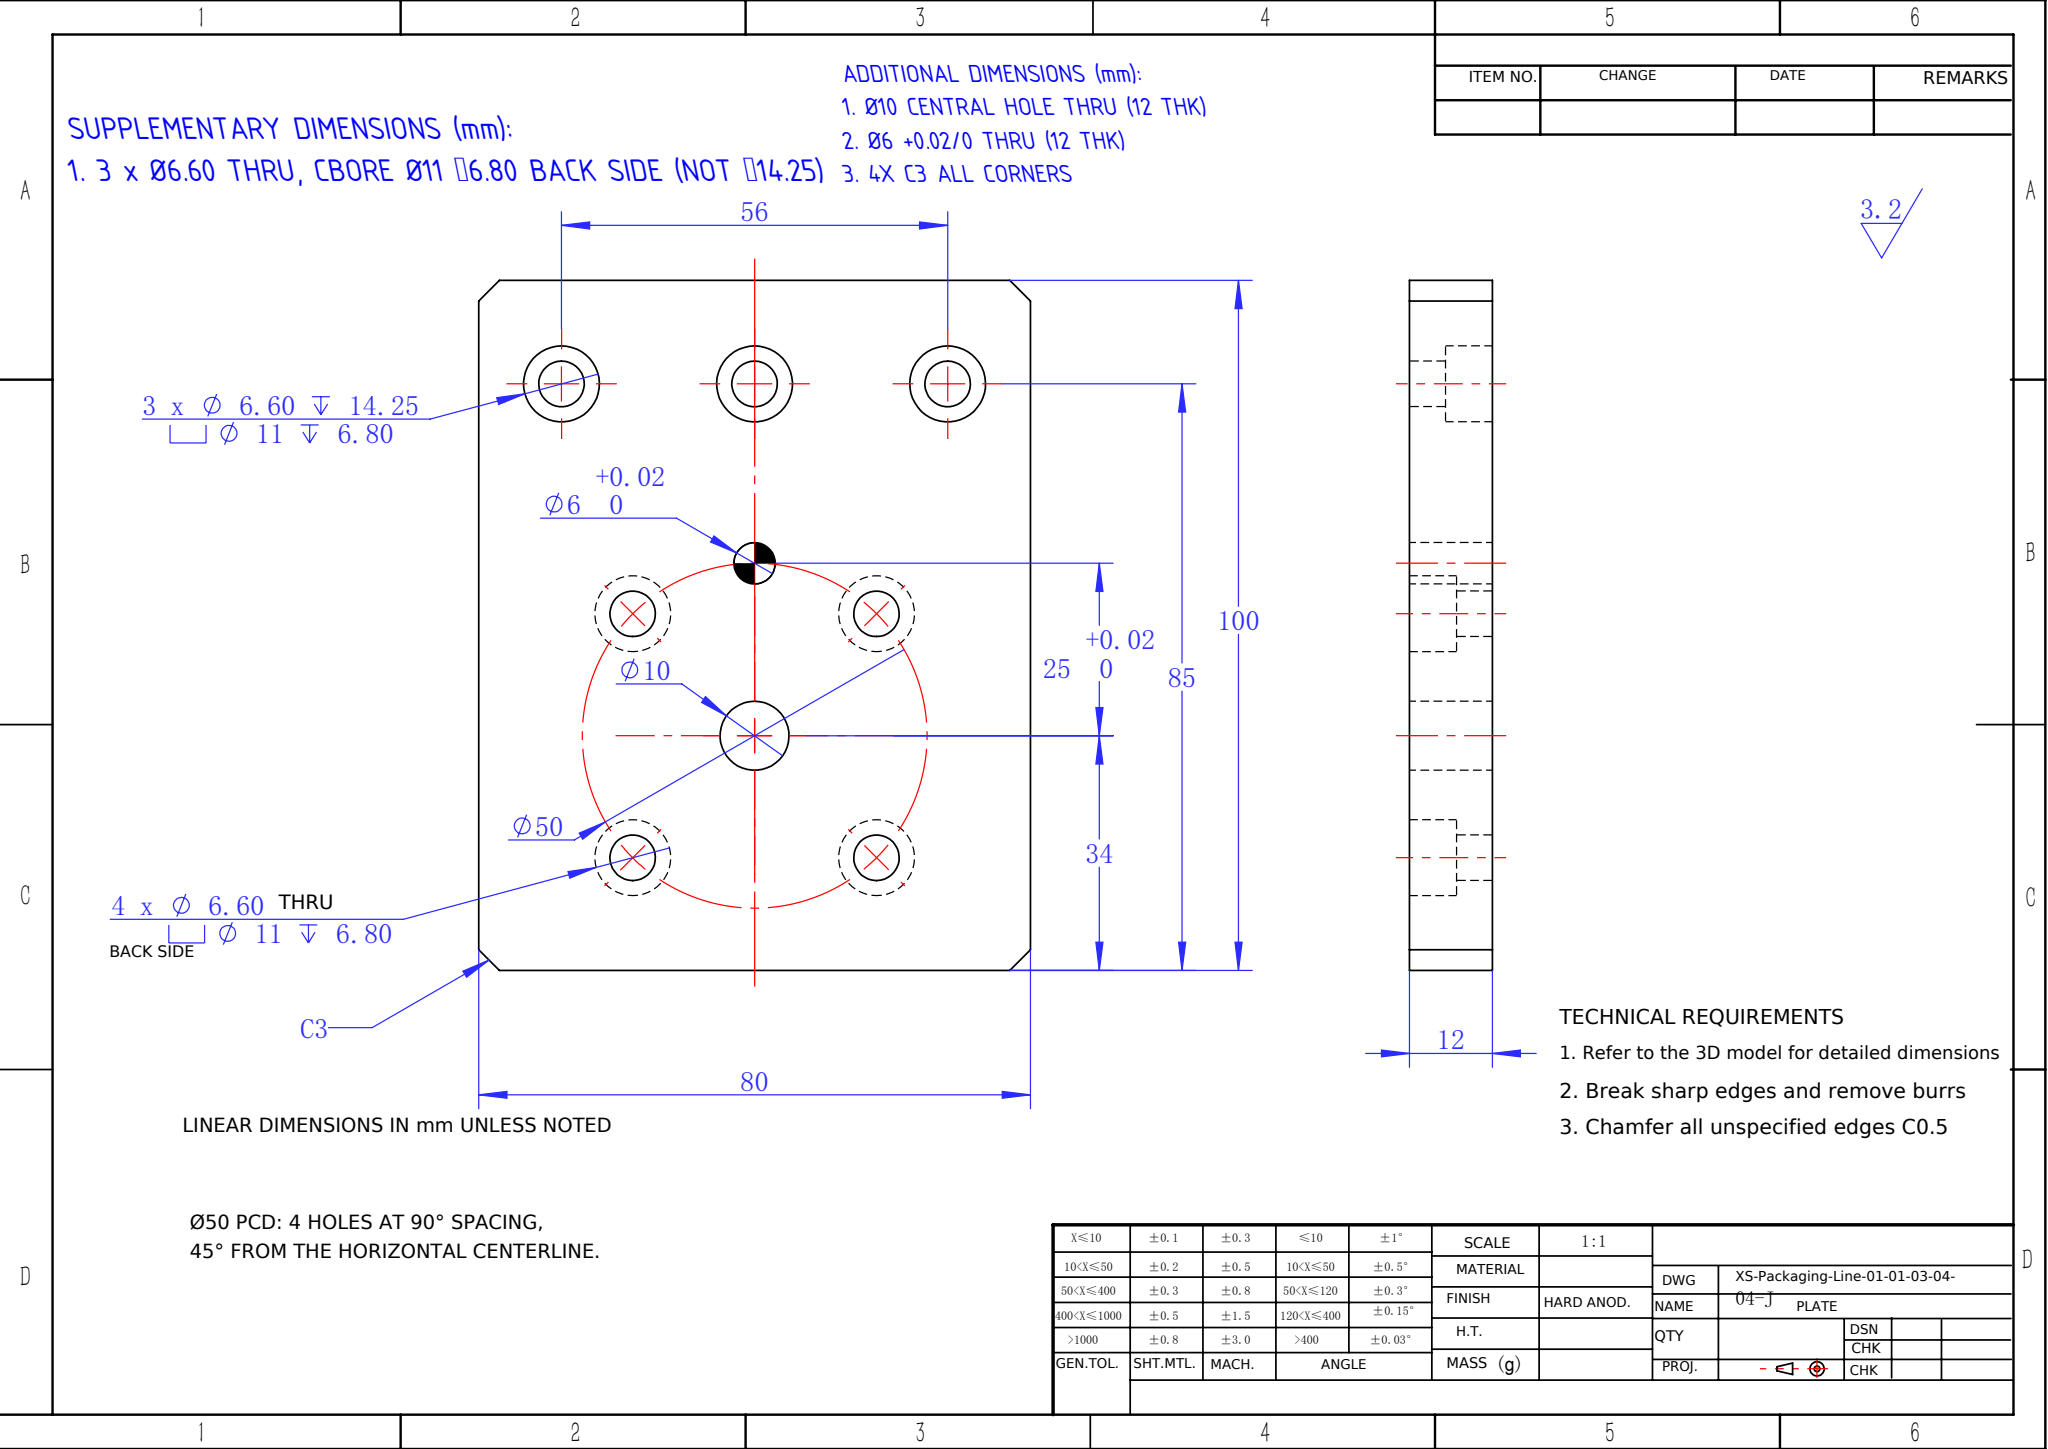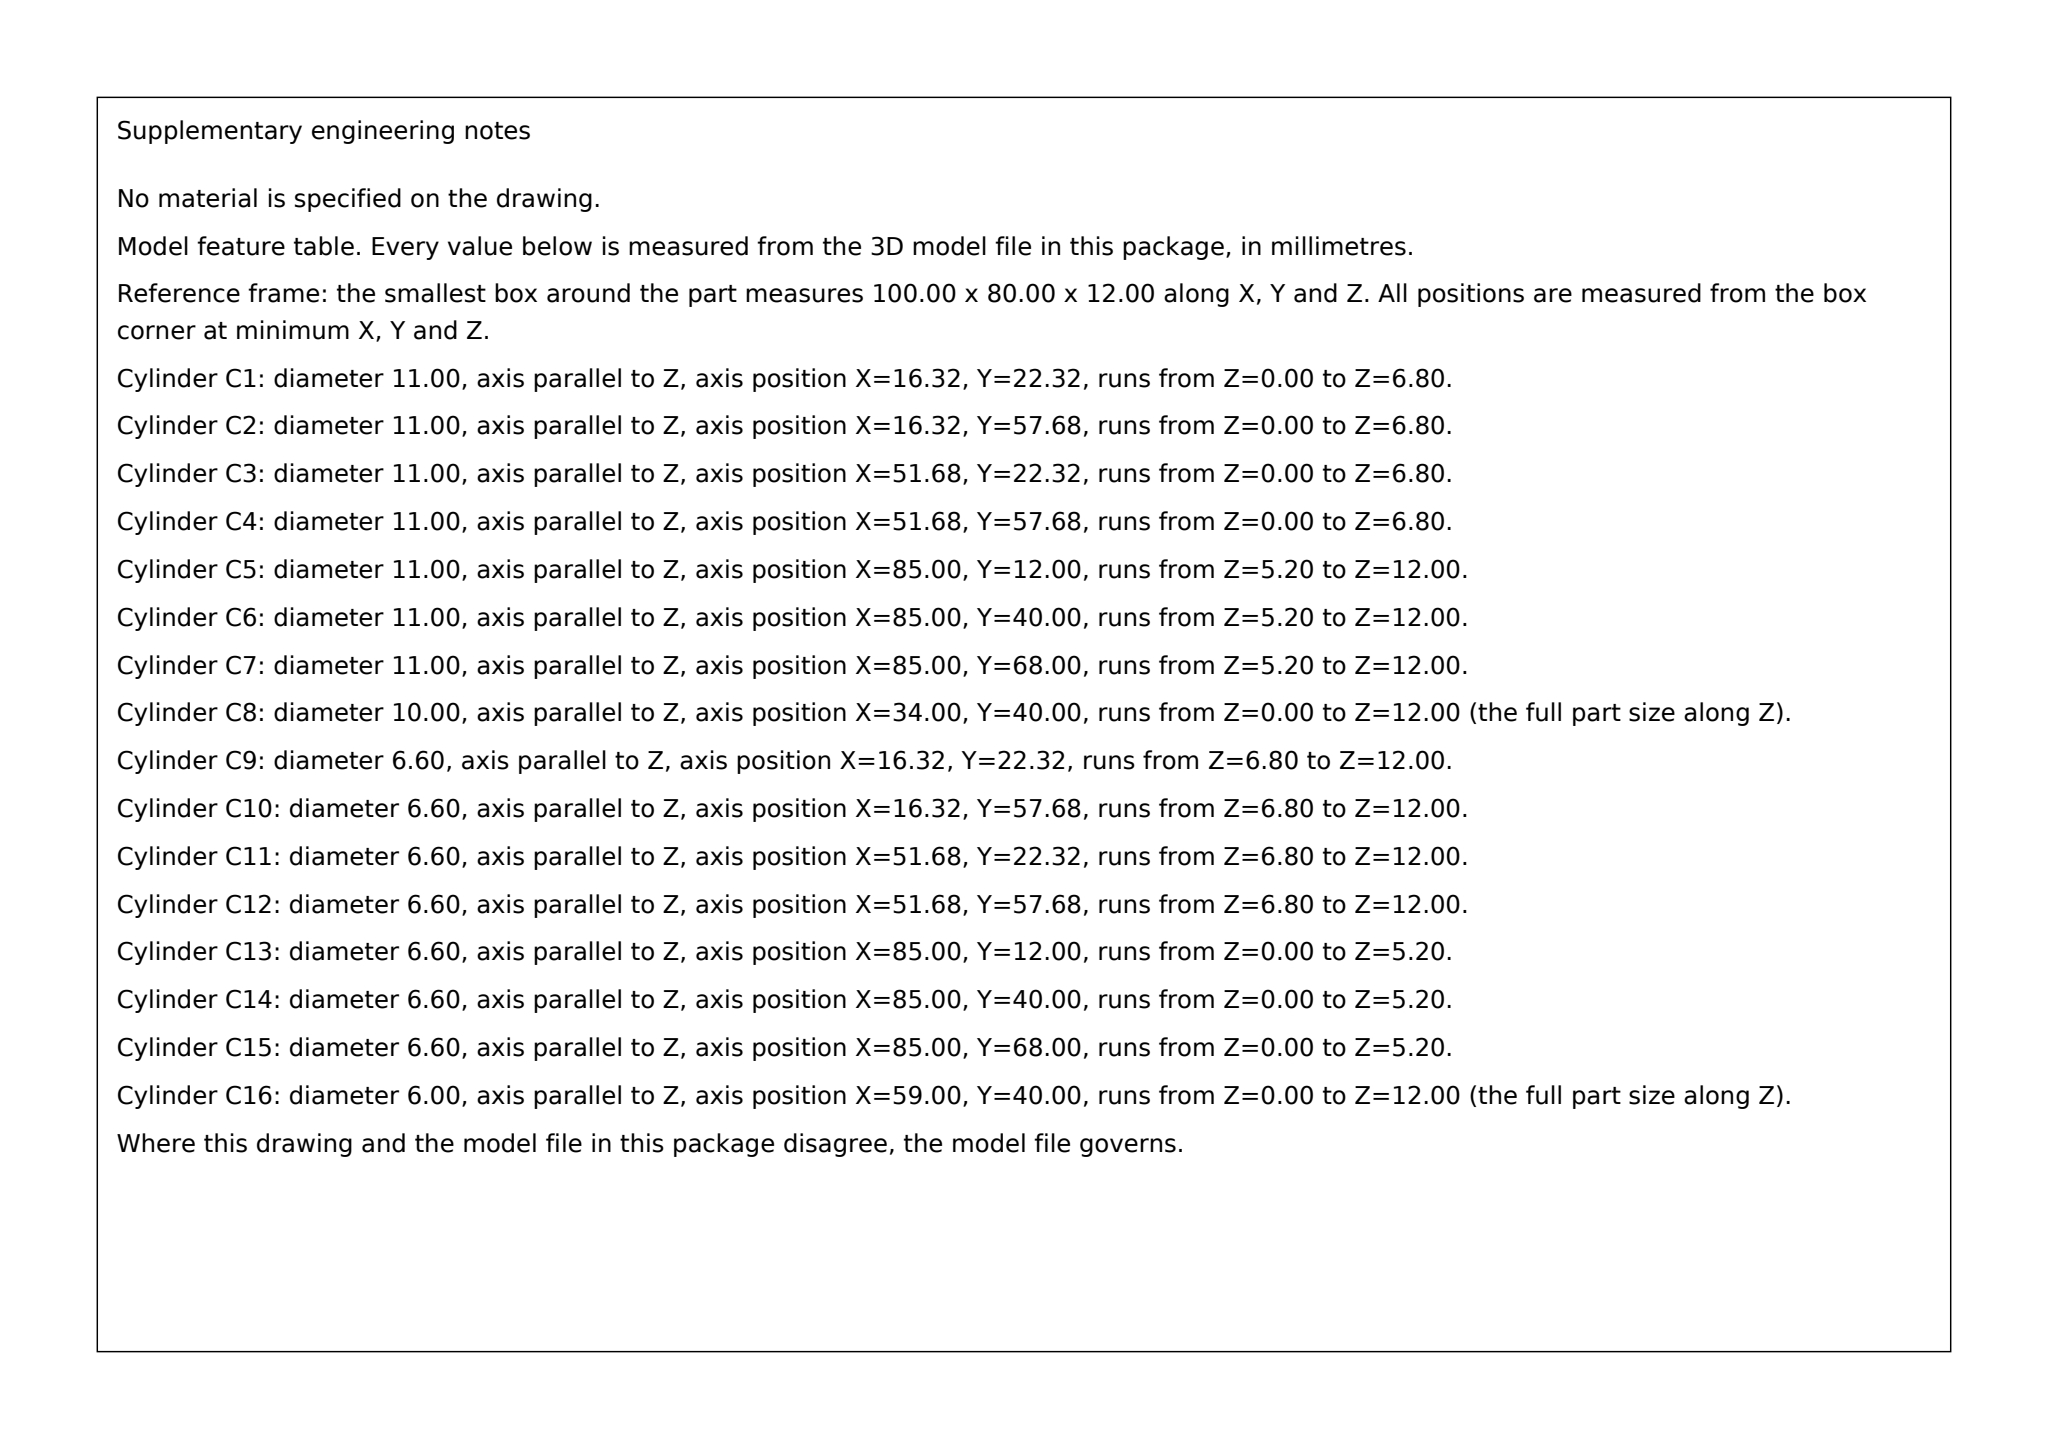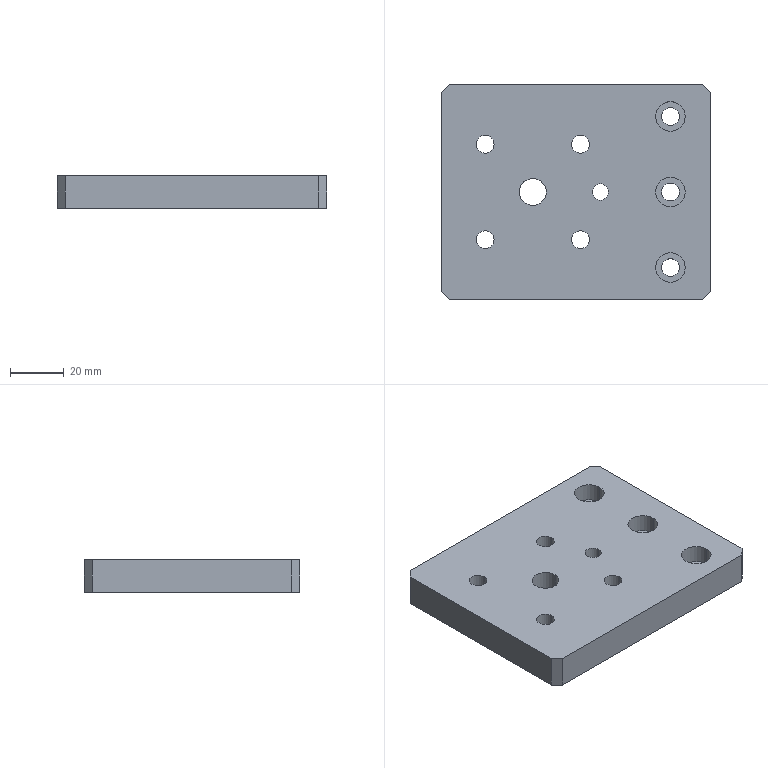Part | SolidWorks | mm | 1 solid | 49 faces | box 100 x 80 x 12 mm | volume 88733 mm3 | cylinder 32 | plane 17 | commonest cylinder face diameters 11 x14 6.6 x14 6 x2 10 x2
build123d program:
from build123d import *

# Parameters (mm, degrees)
SKETCH1_W                                       = 100
SKETCH1_H                                       = 80
BOSS_EXTRUDE1_DEPTH                             = 12
CHAMFER1_SIZE                                   = 3
M6_HEX_SOCKET_HEAD_CAP_SCREW_CBORE1_D           = 6.6
M6_HEX_SOCKET_HEAD_CAP_SCREW_CBORE1_DEPTH       = 14.25
M6_HEX_SOCKET_HEAD_CAP_SCREW_CBORE1_CBORE_D     = 11
M6_HEX_SOCKET_HEAD_CAP_SCREW_CBORE1_CBORE_DEPTH = 6.8
M6_HEX_SOCKET_HEAD_CAP_SCREW_CBORE1_TIP         = 1.983
SKETCH6_R                                       = 5
CUT_EXTRUDE1_DEPTH                              = 66.146
M6_HEX_SOCKET_HEAD_CAP_SCREW_CBORE2_D           = 6.6
M6_HEX_SOCKET_HEAD_CAP_SCREW_CBORE2_CBORE_D     = 11
M6_HEX_SOCKET_HEAD_CAP_SCREW_CBORE2_CBORE_DEPTH = 6.8
F_6_0MM_DOWEL_PIN_HOLE1_D                       = 6


with BuildPart() as part:
    # Sketch1 → Boss-Extrude1 (new body)
    with BuildSketch(Plane.XY):
        Rectangle(SKETCH1_W, SKETCH1_H)
    extrude(amount=BOSS_EXTRUDE1_DEPTH)

    # Chamfer1
    chamfer1_edges = [part.edges().sort_by_distance(p)[0] for p in [
        (50, -40, 6),
        (-50, -40, 6),
        (-50, 40, 6),
        (50, 40, 6),
    ]]
    chamfer(chamfer1_edges, length=CHAMFER1_SIZE)

    # M6 Hex Socket Head Cap Screw CBORE1
    with Locations(Plane.XY.offset(12)):
        with Locations((35, 28), (35, -28), (35, 0)):
            CounterBoreHole(M6_HEX_SOCKET_HEAD_CAP_SCREW_CBORE1_D / 2, M6_HEX_SOCKET_HEAD_CAP_SCREW_CBORE1_CBORE_D / 2, M6_HEX_SOCKET_HEAD_CAP_SCREW_CBORE1_CBORE_DEPTH, depth=M6_HEX_SOCKET_HEAD_CAP_SCREW_CBORE1_DEPTH)
            with Locations((0, 0, -(M6_HEX_SOCKET_HEAD_CAP_SCREW_CBORE1_DEPTH + M6_HEX_SOCKET_HEAD_CAP_SCREW_CBORE1_TIP / 2))):  # 118° drill point
                Cone(0, M6_HEX_SOCKET_HEAD_CAP_SCREW_CBORE1_D / 2, M6_HEX_SOCKET_HEAD_CAP_SCREW_CBORE1_TIP, mode=Mode.SUBTRACT)

    # Sketch6 → Cut-Extrude1 (cut, through all)
    with BuildSketch(Plane.XY.offset(12)):
        with Locations((-16, 0)):
            Circle(SKETCH6_R)
    extrude(amount=-CUT_EXTRUDE1_DEPTH, mode=Mode.SUBTRACT)

    # M6 Hex Socket Head Cap Screw CBORE2 (through all)
    with Locations(Plane(origin=(0, 0, 0), x_dir=(-1, 0, 0), z_dir=(0, 0, -1))):
        with Locations((33.678, 17.678), (33.678, -17.678), (-1.678, -17.678), (-1.678, 17.678)):
            CounterBoreHole(M6_HEX_SOCKET_HEAD_CAP_SCREW_CBORE2_D / 2, M6_HEX_SOCKET_HEAD_CAP_SCREW_CBORE2_CBORE_D / 2, M6_HEX_SOCKET_HEAD_CAP_SCREW_CBORE2_CBORE_DEPTH)

    # 6.0mm Dowel Pin Hole1 (through all)
    with Locations(Plane(origin=(0, 0, 0), x_dir=(-1, 0, 0), z_dir=(0, 0, -1))):
        with Locations((-9, 0)):
            Hole(F_6_0MM_DOWEL_PIN_HOLE1_D / 2)


solid = part.part